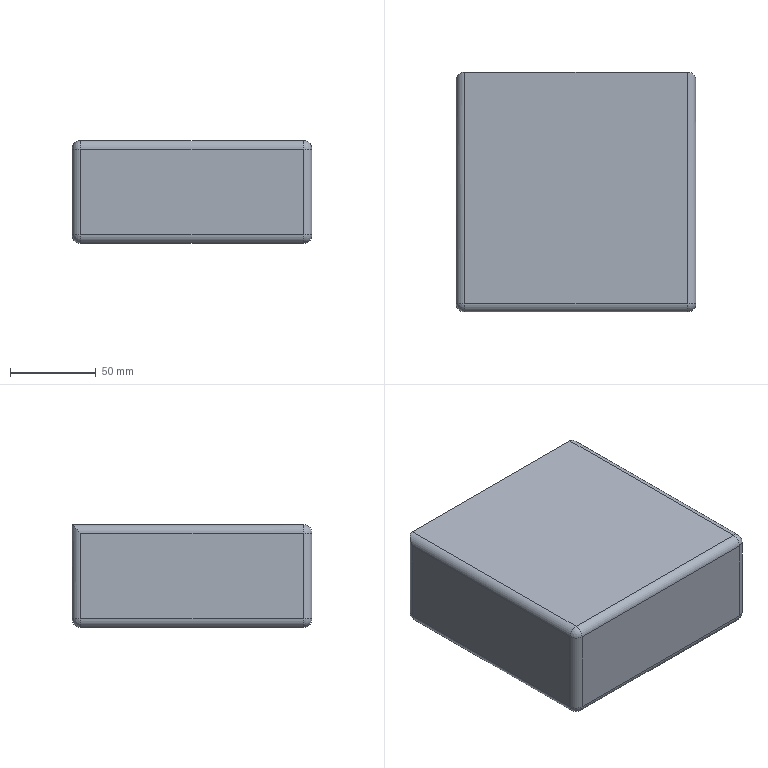Component | SolidWorks | ConnectingBlock-1 | 1 solid | 26 faces | box 140 x 140 x 60 mm | volume 1078498 mm3 | cylinder 13 | plane 7 | sphere 6 | commonest cylinder face diameters 10 x11 60 x2
build123d program:
from build123d import *

# Parameters (mm, degrees)
SKETCH1_W                 = 140
SKETCH1_H                 = 140
BOSS_EXTRUDE1_DEPTH       = 60
FILLET1_R                 = 5
SKETCH2_R                 = 30
REPAIR_RODENDSOCKET_DEPTH = 16.832


with BuildPart() as part:
    # Sketch1 → Boss-Extrude1 (new body)
    with BuildSketch(Plane(origin=(0, 0, -32.222), x_dir=(-1, 0, 0), z_dir=(0, 0, -1))):
        Rectangle(SKETCH1_W, SKETCH1_H)
    extrude(amount=-BOSS_EXTRUDE1_DEPTH)

    # Fillet1
    fillet1_edges = [part.edges().sort_by_distance(p)[0] for p in [
        (0, -70, 27.778),
        (-70, 0, 27.778),
        (0, -70, -32.222),
        (70, 0, -32.222),
        (0, 70, -32.222),
        (-70, 0, -32.222),
        (-70, -70, -2.222),
        (70, -70, -2.222),
        (70, 70, -2.222),
        (-70, 70, -2.222),
        (0, 70, 27.778),
    ]]
    fillet(fillet1_edges, radius=FILLET1_R)

    # Sketch2 → Repair_RodEndSocket (cut, symmetric)
    with BuildSketch(Plane.XY.offset(-16.832)):
        with Locations((0, 0)):
            Circle(SKETCH2_R)
    extrude(amount=REPAIR_RODENDSOCKET_DEPTH, both=True, mode=Mode.SUBTRACT)


solid = part.part

# Placed as in the assembly
solid = solid.moved(Location((-505.158, 870.769, 981.663), (0, 0, 90)))
STEP:
#1=CARTESIAN_POINT('',(-19.888,35.463,37.38));
#2=VERTEX_POINT('',#1);
#3=CARTESIAN_POINT('',(-19.888,33.101,37.38));
#4=VERTEX_POINT('',#3);
#5=CARTESIAN_POINT('',(-19.888,34.282,37.38));
#6=DIRECTION('',(0.,0.,-1.));
#7=DIRECTION('',(0.,-1.,0.));
#8=AXIS2_PLACEMENT_3D('',#5,#6,#7);
#9=CIRCLE('',#8,1.181);
#10=EDGE_CURVE('',#2,#4,#9,.T.);
#11=ORIENTED_EDGE('',*,*,#10,.T.);
#12=CARTESIAN_POINT('',(-19.888,33.101,38.648));
#13=VERTEX_POINT('',#12);
#14=CARTESIAN_POINT('',(-19.888,33.101,37.323));
#15=DIRECTION('',(0.,0.,1.));
#16=VECTOR('',#15,39.37);
#17=LINE('',#14,#16);
#18=EDGE_CURVE('',#4,#13,#17,.T.);
#19=ORIENTED_EDGE('',*,*,#18,.T.);
#20=CARTESIAN_POINT('',(-19.888,35.463,38.648));
#21=VERTEX_POINT('',#20);
#22=CARTESIAN_POINT('',(-19.888,34.282,38.648));
#23=DIRECTION('',(0.,0.,1.));
#24=DIRECTION('',(0.,1.,0.));
#25=AXIS2_PLACEMENT_3D('',#22,#23,#24);
#26=CIRCLE('',#25,1.181);
#27=EDGE_CURVE('',#13,#21,#26,.T.);
#28=ORIENTED_EDGE('',*,*,#27,.T.);
#29=CARTESIAN_POINT('',(-19.888,35.463,37.323));
#30=DIRECTION('',(0.,0.,1.));
#31=VECTOR('',#30,39.37);
#32=LINE('',#29,#31);
#33=EDGE_CURVE('',#2,#21,#32,.T.);
#34=ORIENTED_EDGE('',*,*,#33,.F.);
#35=EDGE_LOOP('',(#11,#19,#28,#34));
#36=FACE_OUTER_BOUND('',#35,.T.);
#37=CARTESIAN_POINT('',(-19.888,34.282,37.323));
#38=DIRECTION('',(0.,0.,1.));
#39=DIRECTION('',(0.,1.,0.));
#40=AXIS2_PLACEMENT_3D('',#37,#38,#39);
#41=CYLINDRICAL_SURFACE('',#40,1.181);
#42=ADVANCED_FACE('',(#36),#41,.F.);
#43=CARTESIAN_POINT('',(-22.447,31.526,37.576));
#44=VERTEX_POINT('',#43);
#45=CARTESIAN_POINT('',(-17.329,31.526,37.576));
#46=VERTEX_POINT('',#45);
#47=CARTESIAN_POINT('',(-17.132,31.526,37.576));
#48=DIRECTION('',(1.,0.,0.));
#49=VECTOR('',#48,39.37);
#50=LINE('',#47,#49);
#51=EDGE_CURVE('',#44,#46,#50,.T.);
#52=ORIENTED_EDGE('',*,*,#51,.T.);
#53=CARTESIAN_POINT('',(-17.329,31.526,39.545));
#54=VERTEX_POINT('',#53);
#55=CARTESIAN_POINT('',(-17.329,31.526,39.742));
#56=DIRECTION('',(0.,0.,1.));
#57=VECTOR('',#56,39.37);
#58=LINE('',#55,#57);
#59=EDGE_CURVE('',#46,#54,#58,.T.);
#60=ORIENTED_EDGE('',*,*,#59,.T.);
#61=CARTESIAN_POINT('',(-22.447,31.526,39.545));
#62=VERTEX_POINT('',#61);
#63=CARTESIAN_POINT('',(-22.644,31.526,39.545));
#64=DIRECTION('',(-1.,0.,0.));
#65=VECTOR('',#64,39.37);
#66=LINE('',#63,#65);
#67=EDGE_CURVE('',#54,#62,#66,.T.);
#68=ORIENTED_EDGE('',*,*,#67,.T.);
#69=CARTESIAN_POINT('',(-22.447,31.526,39.742));
#70=DIRECTION('',(0.,0.,-1.));
#71=VECTOR('',#70,39.37);
#72=LINE('',#69,#71);
#73=EDGE_CURVE('',#62,#44,#72,.T.);
#74=ORIENTED_EDGE('',*,*,#73,.T.);
#75=EDGE_LOOP('',(#52,#60,#68,#74));
#76=FACE_OUTER_BOUND('',#75,.T.);
#77=CARTESIAN_POINT('',(-17.132,31.526,39.742));
#78=DIRECTION('',(0.,-1.,0.));
#79=DIRECTION('',(0.,0.,1.));
#80=AXIS2_PLACEMENT_3D('',#77,#78,#79);
#81=PLANE('',#80);
#82=ADVANCED_FACE('',(#76),#81,.T.);
#83=CARTESIAN_POINT('',(-17.132,36.841,37.576));
#84=VERTEX_POINT('',#83);
#85=CARTESIAN_POINT('',(-17.132,36.841,39.545));
#86=VERTEX_POINT('',#85);
#87=CARTESIAN_POINT('',(-17.132,36.841,39.742));
#88=DIRECTION('',(0.,0.,1.));
#89=VECTOR('',#88,39.37);
#90=LINE('',#87,#89);
#91=EDGE_CURVE('',#84,#86,#90,.T.);
#92=ORIENTED_EDGE('',*,*,#91,.T.);
#93=CARTESIAN_POINT('',(-17.132,31.723,39.545));
#94=VERTEX_POINT('',#93);
#95=CARTESIAN_POINT('',(-17.132,31.526,39.545));
#96=DIRECTION('',(0.,-1.,0.));
#97=VECTOR('',#96,39.37);
#98=LINE('',#95,#97);
#99=EDGE_CURVE('',#86,#94,#98,.T.);
#100=ORIENTED_EDGE('',*,*,#99,.T.);
#101=CARTESIAN_POINT('',(-17.132,31.723,37.576));
#102=VERTEX_POINT('',#101);
#103=CARTESIAN_POINT('',(-17.132,31.723,39.742));
#104=DIRECTION('',(0.,0.,-1.));
#105=VECTOR('',#104,39.37);
#106=LINE('',#103,#105);
#107=EDGE_CURVE('',#94,#102,#106,.T.);
#108=ORIENTED_EDGE('',*,*,#107,.T.);
#109=CARTESIAN_POINT('',(-17.132,37.038,37.576));
#110=DIRECTION('',(0.,1.,0.));
#111=VECTOR('',#110,39.37);
#112=LINE('',#109,#111);
#113=EDGE_CURVE('',#102,#84,#112,.T.);
#114=ORIENTED_EDGE('',*,*,#113,.T.);
#115=EDGE_LOOP('',(#92,#100,#108,#114));
#116=FACE_OUTER_BOUND('',#115,.T.);
#117=CARTESIAN_POINT('',(-17.132,37.038,39.742));
#118=DIRECTION('',(1.,0.,0.));
#119=DIRECTION('',(0.,0.,-1.));
#120=AXIS2_PLACEMENT_3D('',#117,#118,#119);
#121=PLANE('',#120);
#122=ADVANCED_FACE('',(#116),#121,.T.);
#123=CARTESIAN_POINT('',(-22.447,37.038,39.742));
#124=VERTEX_POINT('',#123);
#125=CARTESIAN_POINT('',(-17.329,37.038,39.742));
#126=VERTEX_POINT('',#125);
#127=CARTESIAN_POINT('',(-22.644,37.038,39.742));
#128=DIRECTION('',(1.,0.,0.));
#129=VECTOR('',#128,39.37);
#130=LINE('',#127,#129);
#131=EDGE_CURVE('',#124,#126,#130,.T.);
#132=ORIENTED_EDGE('',*,*,#131,.T.);
#133=CARTESIAN_POINT('',(-17.329,37.038,37.576));
#134=VERTEX_POINT('',#133);
#135=CARTESIAN_POINT('',(-17.329,37.038,39.742));
#136=DIRECTION('',(0.,0.,-1.));
#137=VECTOR('',#136,39.37);
#138=LINE('',#135,#137);
#139=EDGE_CURVE('',#126,#134,#138,.T.);
#140=ORIENTED_EDGE('',*,*,#139,.T.);
#141=CARTESIAN_POINT('',(-22.447,37.038,37.576));
#142=VERTEX_POINT('',#141);
#143=CARTESIAN_POINT('',(-22.644,37.038,37.576));
#144=DIRECTION('',(-1.,0.,0.));
#145=VECTOR('',#144,39.37);
#146=LINE('',#143,#145);
#147=EDGE_CURVE('',#134,#142,#146,.T.);
#148=ORIENTED_EDGE('',*,*,#147,.T.);
#149=CARTESIAN_POINT('',(-22.447,37.038,39.742));
#150=DIRECTION('',(0.,0.,1.));
#151=VECTOR('',#150,39.37);
#152=LINE('',#149,#151);
#153=EDGE_CURVE('',#142,#124,#152,.T.);
#154=ORIENTED_EDGE('',*,*,#153,.T.);
#155=EDGE_LOOP('',(#132,#140,#148,#154));
#156=FACE_OUTER_BOUND('',#155,.T.);
#157=CARTESIAN_POINT('',(-22.644,37.038,39.742));
#158=DIRECTION('',(0.,1.,0.));
#159=DIRECTION('',(0.,0.,-1.));
#160=AXIS2_PLACEMENT_3D('',#157,#158,#159);
#161=PLANE('',#160);
#162=ADVANCED_FACE('',(#156),#161,.T.);
#163=CARTESIAN_POINT('',(-22.644,36.841,37.576));
#164=VERTEX_POINT('',#163);
#165=CARTESIAN_POINT('',(-22.644,31.723,37.576));
#166=VERTEX_POINT('',#165);
#167=CARTESIAN_POINT('',(-22.644,31.526,37.576));
#168=DIRECTION('',(0.,-1.,0.));
#169=VECTOR('',#168,39.37);
#170=LINE('',#167,#169);
#171=EDGE_CURVE('',#164,#166,#170,.T.);
#172=ORIENTED_EDGE('',*,*,#171,.T.);
#173=CARTESIAN_POINT('',(-22.644,31.723,39.545));
#174=VERTEX_POINT('',#173);
#175=CARTESIAN_POINT('',(-22.644,31.723,39.742));
#176=DIRECTION('',(0.,0.,1.));
#177=VECTOR('',#176,39.37);
#178=LINE('',#175,#177);
#179=EDGE_CURVE('',#166,#174,#178,.T.);
#180=ORIENTED_EDGE('',*,*,#179,.T.);
#181=CARTESIAN_POINT('',(-22.644,36.841,39.545));
#182=VERTEX_POINT('',#181);
#183=CARTESIAN_POINT('',(-22.644,37.038,39.545));
#184=DIRECTION('',(0.,1.,0.));
#185=VECTOR('',#184,39.37);
#186=LINE('',#183,#185);
#187=EDGE_CURVE('',#174,#182,#186,.T.);
#188=ORIENTED_EDGE('',*,*,#187,.T.);
#189=CARTESIAN_POINT('',(-22.644,36.841,39.742));
#190=DIRECTION('',(0.,0.,-1.));
#191=VECTOR('',#190,39.37);
#192=LINE('',#189,#191);
#193=EDGE_CURVE('',#182,#164,#192,.T.);
#194=ORIENTED_EDGE('',*,*,#193,.T.);
#195=EDGE_LOOP('',(#172,#180,#188,#194));
#196=FACE_OUTER_BOUND('',#195,.T.);
#197=CARTESIAN_POINT('',(-22.644,31.526,39.742));
#198=DIRECTION('',(-1.,0.,0.));
#199=DIRECTION('',(0.,0.,1.));
#200=AXIS2_PLACEMENT_3D('',#197,#198,#199);
#201=PLANE('',#200);
#202=ADVANCED_FACE('',(#196),#201,.T.);
#203=CARTESIAN_POINT('',(-22.447,31.723,39.742));
#204=VERTEX_POINT('',#203);
#205=CARTESIAN_POINT('',(-17.329,31.723,39.742));
#206=VERTEX_POINT('',#205);
#207=CARTESIAN_POINT('',(-17.132,31.723,39.742));
#208=DIRECTION('',(1.,0.,0.));
#209=VECTOR('',#208,39.37);
#210=LINE('',#207,#209);
#211=EDGE_CURVE('',#204,#206,#210,.T.);
#212=ORIENTED_EDGE('',*,*,#211,.T.);
#213=CARTESIAN_POINT('',(-17.329,37.038,39.742));
#214=DIRECTION('',(0.,1.,0.));
#215=VECTOR('',#214,39.37);
#216=LINE('',#213,#215);
#217=EDGE_CURVE('',#206,#126,#216,.T.);
#218=ORIENTED_EDGE('',*,*,#217,.T.);
#219=ORIENTED_EDGE('',*,*,#131,.F.);
#220=CARTESIAN_POINT('',(-22.447,31.526,39.742));
#221=DIRECTION('',(0.,-1.,0.));
#222=VECTOR('',#221,39.37);
#223=LINE('',#220,#222);
#224=EDGE_CURVE('',#124,#204,#223,.T.);
#225=ORIENTED_EDGE('',*,*,#224,.T.);
#226=EDGE_LOOP('',(#212,#218,#219,#225));
#227=FACE_OUTER_BOUND('',#226,.T.);
#228=CARTESIAN_POINT('',(-19.888,34.282,39.742));
#229=DIRECTION('',(0.,0.,-1.));
#230=DIRECTION('',(0.,-1.,0.));
#231=AXIS2_PLACEMENT_3D('',#228,#229,#230);
#232=PLANE('',#231);
#233=ADVANCED_FACE('',(#227),#232,.F.);
#234=ORIENTED_EDGE('',*,*,#10,.F.);
#235=CARTESIAN_POINT('',(-19.888,34.282,37.38));
#236=DIRECTION('',(0.,0.,-1.));
#237=DIRECTION('',(0.,-1.,0.));
#238=AXIS2_PLACEMENT_3D('',#235,#236,#237);
#239=CIRCLE('',#238,1.181);
#240=EDGE_CURVE('',#4,#2,#239,.T.);
#241=ORIENTED_EDGE('',*,*,#240,.F.);
#242=EDGE_LOOP('',(#234,#241));
#243=FACE_BOUND('',#242,.T.);
#244=CARTESIAN_POINT('',(-22.447,36.841,37.38));
#245=VERTEX_POINT('',#244);
#246=CARTESIAN_POINT('',(-17.329,36.841,37.38));
#247=VERTEX_POINT('',#246);
#248=CARTESIAN_POINT('',(-19.888,36.841,37.38));
#249=DIRECTION('',(1.,0.,0.));
#250=VECTOR('',#249,39.37);
#251=LINE('',#248,#250);
#252=EDGE_CURVE('',#245,#247,#251,.T.);
#253=ORIENTED_EDGE('',*,*,#252,.T.);
#254=CARTESIAN_POINT('',(-17.329,31.723,37.38));
#255=VERTEX_POINT('',#254);
#256=CARTESIAN_POINT('',(-17.329,34.282,37.38));
#257=DIRECTION('',(0.,-1.,0.));
#258=VECTOR('',#257,39.37);
#259=LINE('',#256,#258);
#260=EDGE_CURVE('',#247,#255,#259,.T.);
#261=ORIENTED_EDGE('',*,*,#260,.T.);
#262=CARTESIAN_POINT('',(-22.447,31.723,37.38));
#263=VERTEX_POINT('',#262);
#264=CARTESIAN_POINT('',(-19.888,31.723,37.38));
#265=DIRECTION('',(-1.,0.,0.));
#266=VECTOR('',#265,39.37);
#267=LINE('',#264,#266);
#268=EDGE_CURVE('',#255,#263,#267,.T.);
#269=ORIENTED_EDGE('',*,*,#268,.T.);
#270=CARTESIAN_POINT('',(-22.447,34.282,37.38));
#271=DIRECTION('',(0.,1.,0.));
#272=VECTOR('',#271,39.37);
#273=LINE('',#270,#272);
#274=EDGE_CURVE('',#263,#245,#273,.T.);
#275=ORIENTED_EDGE('',*,*,#274,.T.);
#276=EDGE_LOOP('',(#253,#261,#269,#275));
#277=FACE_OUTER_BOUND('',#276,.T.);
#278=CARTESIAN_POINT('',(-19.888,34.282,37.38));
#279=DIRECTION('',(0.,0.,-1.));
#280=DIRECTION('',(0.,-1.,0.));
#281=AXIS2_PLACEMENT_3D('',#278,#279,#280);
#282=PLANE('',#281);
#283=ADVANCED_FACE('',(#243,#277),#282,.T.);
#284=CARTESIAN_POINT('',(-22.447,31.723,37.576));
#285=DIRECTION('',(0.,-1.,0.));
#286=DIRECTION('',(0.,0.,1.));
#287=AXIS2_PLACEMENT_3D('',#284,#285,#286);
#288=CIRCLE('',#287,0.1969);
#289=EDGE_CURVE('',#166,#263,#288,.T.);
#290=ORIENTED_EDGE('',*,*,#289,.F.);
#291=ORIENTED_EDGE('',*,*,#171,.F.);
#292=CARTESIAN_POINT('',(-22.447,36.841,37.576));
#293=DIRECTION('',(0.,1.,0.));
#294=DIRECTION('',(0.,0.,-1.));
#295=AXIS2_PLACEMENT_3D('',#292,#293,#294);
#296=CIRCLE('',#295,0.1969);
#297=EDGE_CURVE('',#245,#164,#296,.T.);
#298=ORIENTED_EDGE('',*,*,#297,.F.);
#299=ORIENTED_EDGE('',*,*,#274,.F.);
#300=EDGE_LOOP('',(#290,#291,#298,#299));
#301=FACE_OUTER_BOUND('',#300,.T.);
#302=CARTESIAN_POINT('',(-22.447,34.282,37.576));
#303=DIRECTION('',(0.,1.,0.));
#304=DIRECTION('',(0.,0.,-1.));
#305=AXIS2_PLACEMENT_3D('',#302,#303,#304);
#306=CYLINDRICAL_SURFACE('',#305,0.1969);
#307=ADVANCED_FACE('',(#301),#306,.T.);
#308=CARTESIAN_POINT('',(-22.447,31.723,37.576));
#309=DIRECTION('',(0.,0.,1.));
#310=DIRECTION('',(0.,-1.,0.));
#311=AXIS2_PLACEMENT_3D('',#308,#309,#310);
#312=CIRCLE('',#311,0.1969);
#313=EDGE_CURVE('',#166,#44,#312,.T.);
#314=ORIENTED_EDGE('',*,*,#313,.F.);
#315=ORIENTED_EDGE('',*,*,#289,.T.);
#316=CARTESIAN_POINT('',(-22.447,31.723,37.576));
#317=DIRECTION('',(1.,0.,0.));
#318=DIRECTION('',(0.,0.,1.));
#319=AXIS2_PLACEMENT_3D('',#316,#317,#318);
#320=CIRCLE('',#319,0.1969);
#321=EDGE_CURVE('',#44,#263,#320,.T.);
#322=ORIENTED_EDGE('',*,*,#321,.F.);
#323=EDGE_LOOP('',(#314,#315,#322));
#324=FACE_OUTER_BOUND('',#323,.T.);
#325=CARTESIAN_POINT('',(-22.447,31.723,37.576));
#326=DIRECTION('',(-1.,0.,0.));
#327=DIRECTION('',(0.,1.,0.));
#328=AXIS2_PLACEMENT_3D('',#325,#326,#327);
#329=SPHERICAL_SURFACE('',#328,0.1969);
#330=ADVANCED_FACE('',(#324),#329,.T.);
#331=CARTESIAN_POINT('',(-22.447,36.841,37.576));
#332=DIRECTION('',(0.,0.,-1.));
#333=DIRECTION('',(0.,-1.,0.));
#334=AXIS2_PLACEMENT_3D('',#331,#332,#333);
#335=CIRCLE('',#334,0.1969);
#336=EDGE_CURVE('',#164,#142,#335,.T.);
#337=ORIENTED_EDGE('',*,*,#336,.F.);
#338=ORIENTED_EDGE('',*,*,#193,.F.);
#339=CARTESIAN_POINT('',(-22.447,37.038,39.742));
#340=CARTESIAN_POINT('',(-22.562,37.038,39.742));
#341=CARTESIAN_POINT('',(-22.644,36.957,39.66));
#342=CARTESIAN_POINT('',(-22.644,36.841,39.545));
#343=(BOUNDED_CURVE()B_SPLINE_CURVE(3,(#339,#340,#341,#342),.UNSPECIFIED.,.F.,.F.)B_SPLINE_CURVE_WITH_KNOTS((4,4),(3.142,4.712),.UNSPECIFIED.)CURVE()GEOMETRIC_REPRESENTATION_ITEM()RATIONAL_B_SPLINE_CURVE((1.,0.8047,0.8047,1.))REPRESENTATION_ITEM(''));
#344=EDGE_CURVE('',#124,#182,#343,.T.);
#345=ORIENTED_EDGE('',*,*,#344,.F.);
#346=ORIENTED_EDGE('',*,*,#153,.F.);
#347=EDGE_LOOP('',(#337,#338,#345,#346));
#348=FACE_OUTER_BOUND('',#347,.T.);
#349=CARTESIAN_POINT('',(-22.447,36.841,39.742));
#350=DIRECTION('',(0.,0.,-1.));
#351=DIRECTION('',(0.,-1.,0.));
#352=AXIS2_PLACEMENT_3D('',#349,#350,#351);
#353=CYLINDRICAL_SURFACE('',#352,0.1969);
#354=ADVANCED_FACE('',(#348),#353,.T.);
#355=ORIENTED_EDGE('',*,*,#297,.T.);
#356=ORIENTED_EDGE('',*,*,#336,.T.);
#357=CARTESIAN_POINT('',(-22.447,36.841,37.576));
#358=DIRECTION('',(1.,0.,0.));
#359=DIRECTION('',(0.,0.,1.));
#360=AXIS2_PLACEMENT_3D('',#357,#358,#359);
#361=CIRCLE('',#360,0.1969);
#362=EDGE_CURVE('',#245,#142,#361,.T.);
#363=ORIENTED_EDGE('',*,*,#362,.F.);
#364=EDGE_LOOP('',(#355,#356,#363));
#365=FACE_OUTER_BOUND('',#364,.T.);
#366=CARTESIAN_POINT('',(-22.447,36.841,37.576));
#367=DIRECTION('',(-1.,0.,0.));
#368=DIRECTION('',(0.,1.,0.));
#369=AXIS2_PLACEMENT_3D('',#366,#367,#368);
#370=SPHERICAL_SURFACE('',#369,0.1969);
#371=ADVANCED_FACE('',(#365),#370,.T.);
#372=ORIENTED_EDGE('',*,*,#321,.T.);
#373=ORIENTED_EDGE('',*,*,#268,.F.);
#374=CARTESIAN_POINT('',(-17.329,31.723,37.576));
#375=DIRECTION('',(1.,0.,0.));
#376=DIRECTION('',(0.,0.,-1.));
#377=AXIS2_PLACEMENT_3D('',#374,#375,#376);
#378=CIRCLE('',#377,0.1969);
#379=EDGE_CURVE('',#46,#255,#378,.T.);
#380=ORIENTED_EDGE('',*,*,#379,.F.);
#381=ORIENTED_EDGE('',*,*,#51,.F.);
#382=EDGE_LOOP('',(#372,#373,#380,#381));
#383=FACE_OUTER_BOUND('',#382,.T.);
#384=CARTESIAN_POINT('',(-19.888,31.723,37.576));
#385=DIRECTION('',(-1.,0.,0.));
#386=DIRECTION('',(0.,0.,1.));
#387=AXIS2_PLACEMENT_3D('',#384,#385,#386);
#388=CYLINDRICAL_SURFACE('',#387,0.1969);
#389=ADVANCED_FACE('',(#383),#388,.T.);
#390=ORIENTED_EDGE('',*,*,#313,.T.);
#391=ORIENTED_EDGE('',*,*,#73,.F.);
#392=CARTESIAN_POINT('',(-22.447,31.723,39.545));
#393=DIRECTION('',(0.,0.,1.));
#394=DIRECTION('',(0.,1.,0.));
#395=AXIS2_PLACEMENT_3D('',#392,#393,#394);
#396=CIRCLE('',#395,0.1969);
#397=EDGE_CURVE('',#174,#62,#396,.T.);
#398=ORIENTED_EDGE('',*,*,#397,.F.);
#399=ORIENTED_EDGE('',*,*,#179,.F.);
#400=EDGE_LOOP('',(#390,#391,#398,#399));
#401=FACE_OUTER_BOUND('',#400,.T.);
#402=CARTESIAN_POINT('',(-22.447,31.723,39.742));
#403=DIRECTION('',(0.,0.,-1.));
#404=DIRECTION('',(0.,-1.,0.));
#405=AXIS2_PLACEMENT_3D('',#402,#403,#404);
#406=CYLINDRICAL_SURFACE('',#405,0.1969);
#407=ADVANCED_FACE('',(#401),#406,.T.);
#408=ORIENTED_EDGE('',*,*,#344,.T.);
#409=ORIENTED_EDGE('',*,*,#187,.F.);
#410=CARTESIAN_POINT('',(-22.447,31.723,39.545));
#411=DIRECTION('',(0.,-1.,0.));
#412=DIRECTION('',(0.,0.,1.));
#413=AXIS2_PLACEMENT_3D('',#410,#411,#412);
#414=CIRCLE('',#413,0.1969);
#415=EDGE_CURVE('',#204,#174,#414,.T.);
#416=ORIENTED_EDGE('',*,*,#415,.F.);
#417=ORIENTED_EDGE('',*,*,#224,.F.);
#418=EDGE_LOOP('',(#408,#409,#416,#417));
#419=FACE_OUTER_BOUND('',#418,.T.);
#420=CARTESIAN_POINT('',(-22.447,31.526,39.545));
#421=DIRECTION('',(0.,-1.,0.));
#422=DIRECTION('',(0.,0.,1.));
#423=AXIS2_PLACEMENT_3D('',#420,#421,#422);
#424=CYLINDRICAL_SURFACE('',#423,0.1969);
#425=ADVANCED_FACE('',(#419),#424,.T.);
#426=ORIENTED_EDGE('',*,*,#362,.T.);
#427=ORIENTED_EDGE('',*,*,#147,.F.);
#428=CARTESIAN_POINT('',(-17.329,36.841,37.576));
#429=DIRECTION('',(1.,0.,0.));
#430=DIRECTION('',(0.,0.,-1.));
#431=AXIS2_PLACEMENT_3D('',#428,#429,#430);
#432=CIRCLE('',#431,0.1969);
#433=EDGE_CURVE('',#247,#134,#432,.T.);
#434=ORIENTED_EDGE('',*,*,#433,.F.);
#435=ORIENTED_EDGE('',*,*,#252,.F.);
#436=EDGE_LOOP('',(#426,#427,#434,#435));
#437=FACE_OUTER_BOUND('',#436,.T.);
#438=CARTESIAN_POINT('',(-19.888,36.841,37.576));
#439=DIRECTION('',(1.,0.,0.));
#440=DIRECTION('',(0.,0.,-1.));
#441=AXIS2_PLACEMENT_3D('',#438,#439,#440);
#442=CYLINDRICAL_SURFACE('',#441,0.1969);
#443=ADVANCED_FACE('',(#437),#442,.T.);
#444=CARTESIAN_POINT('',(-17.329,31.723,37.576));
#445=DIRECTION('',(0.,-1.,0.));
#446=DIRECTION('',(0.,0.,1.));
#447=AXIS2_PLACEMENT_3D('',#444,#445,#446);
#448=CIRCLE('',#447,0.1969);
#449=EDGE_CURVE('',#255,#102,#448,.T.);
#450=ORIENTED_EDGE('',*,*,#449,.F.);
#451=ORIENTED_EDGE('',*,*,#260,.F.);
#452=CARTESIAN_POINT('',(-17.329,36.841,37.576));
#453=DIRECTION('',(0.,1.,0.));
#454=DIRECTION('',(0.,0.,-1.));
#455=AXIS2_PLACEMENT_3D('',#452,#453,#454);
#456=CIRCLE('',#455,0.1969);
#457=EDGE_CURVE('',#84,#247,#456,.T.);
#458=ORIENTED_EDGE('',*,*,#457,.F.);
#459=ORIENTED_EDGE('',*,*,#113,.F.);
#460=EDGE_LOOP('',(#450,#451,#458,#459));
#461=FACE_OUTER_BOUND('',#460,.T.);
#462=CARTESIAN_POINT('',(-17.329,34.282,37.576));
#463=DIRECTION('',(0.,-1.,0.));
#464=DIRECTION('',(0.,0.,1.));
#465=AXIS2_PLACEMENT_3D('',#462,#463,#464);
#466=CYLINDRICAL_SURFACE('',#465,0.1969);
#467=ADVANCED_FACE('',(#461),#466,.T.);
#468=ORIENTED_EDGE('',*,*,#379,.T.);
#469=ORIENTED_EDGE('',*,*,#449,.T.);
#470=CARTESIAN_POINT('',(-17.329,31.723,37.576));
#471=DIRECTION('',(0.,0.,1.));
#472=DIRECTION('',(0.,-1.,0.));
#473=AXIS2_PLACEMENT_3D('',#470,#471,#472);
#474=CIRCLE('',#473,0.1969);
#475=EDGE_CURVE('',#46,#102,#474,.T.);
#476=ORIENTED_EDGE('',*,*,#475,.F.);
#477=EDGE_LOOP('',(#468,#469,#476));
#478=FACE_OUTER_BOUND('',#477,.T.);
#479=CARTESIAN_POINT('',(-17.329,31.723,37.576));
#480=DIRECTION('',(-1.,0.,0.));
#481=DIRECTION('',(0.,1.,0.));
#482=AXIS2_PLACEMENT_3D('',#479,#480,#481);
#483=SPHERICAL_SURFACE('',#482,0.1969);
#484=ADVANCED_FACE('',(#478),#483,.T.);
#485=ORIENTED_EDGE('',*,*,#415,.T.);
#486=ORIENTED_EDGE('',*,*,#397,.T.);
#487=CARTESIAN_POINT('',(-22.447,31.723,39.545));
#488=DIRECTION('',(1.,0.,0.));
#489=DIRECTION('',(0.,0.,1.));
#490=AXIS2_PLACEMENT_3D('',#487,#488,#489);
#491=CIRCLE('',#490,0.1969);
#492=EDGE_CURVE('',#204,#62,#491,.T.);
#493=ORIENTED_EDGE('',*,*,#492,.F.);
#494=EDGE_LOOP('',(#485,#486,#493));
#495=FACE_OUTER_BOUND('',#494,.T.);
#496=CARTESIAN_POINT('',(-22.447,31.723,39.545));
#497=DIRECTION('',(-1.,0.,0.));
#498=DIRECTION('',(0.,1.,0.));
#499=AXIS2_PLACEMENT_3D('',#496,#497,#498);
#500=SPHERICAL_SURFACE('',#499,0.1969);
#501=ADVANCED_FACE('',(#495),#500,.T.);
#502=ORIENTED_EDGE('',*,*,#457,.T.);
#503=ORIENTED_EDGE('',*,*,#433,.T.);
#504=CARTESIAN_POINT('',(-17.329,36.841,37.576));
#505=DIRECTION('',(0.,0.,1.));
#506=DIRECTION('',(0.,-1.,0.));
#507=AXIS2_PLACEMENT_3D('',#504,#505,#506);
#508=CIRCLE('',#507,0.1969);
#509=EDGE_CURVE('',#84,#134,#508,.T.);
#510=ORIENTED_EDGE('',*,*,#509,.F.);
#511=EDGE_LOOP('',(#502,#503,#510));
#512=FACE_OUTER_BOUND('',#511,.T.);
#513=CARTESIAN_POINT('',(-17.329,36.841,37.576));
#514=DIRECTION('',(-1.,0.,0.));
#515=DIRECTION('',(0.,1.,0.));
#516=AXIS2_PLACEMENT_3D('',#513,#514,#515);
#517=SPHERICAL_SURFACE('',#516,0.1969);
#518=ADVANCED_FACE('',(#512),#517,.T.);
#519=ORIENTED_EDGE('',*,*,#475,.T.);
#520=ORIENTED_EDGE('',*,*,#107,.F.);
#521=CARTESIAN_POINT('',(-17.329,31.723,39.545));
#522=DIRECTION('',(0.,0.,1.));
#523=DIRECTION('',(0.,1.,0.));
#524=AXIS2_PLACEMENT_3D('',#521,#522,#523);
#525=CIRCLE('',#524,0.1969);
#526=EDGE_CURVE('',#54,#94,#525,.T.);
#527=ORIENTED_EDGE('',*,*,#526,.F.);
#528=ORIENTED_EDGE('',*,*,#59,.F.);
#529=EDGE_LOOP('',(#519,#520,#527,#528));
#530=FACE_OUTER_BOUND('',#529,.T.);
#531=CARTESIAN_POINT('',(-17.329,31.723,39.742));
#532=DIRECTION('',(0.,0.,-1.));
#533=DIRECTION('',(0.,-1.,0.));
#534=AXIS2_PLACEMENT_3D('',#531,#532,#533);
#535=CYLINDRICAL_SURFACE('',#534,0.1969);
#536=ADVANCED_FACE('',(#530),#535,.T.);
#537=ORIENTED_EDGE('',*,*,#492,.T.);
#538=ORIENTED_EDGE('',*,*,#67,.F.);
#539=CARTESIAN_POINT('',(-17.329,31.723,39.545));
#540=DIRECTION('',(1.,0.,0.));
#541=DIRECTION('',(0.,0.,-1.));
#542=AXIS2_PLACEMENT_3D('',#539,#540,#541);
#543=CIRCLE('',#542,0.1969);
#544=EDGE_CURVE('',#206,#54,#543,.T.);
#545=ORIENTED_EDGE('',*,*,#544,.F.);
#546=ORIENTED_EDGE('',*,*,#211,.F.);
#547=EDGE_LOOP('',(#537,#538,#545,#546));
#548=FACE_OUTER_BOUND('',#547,.T.);
#549=CARTESIAN_POINT('',(-17.132,31.723,39.545));
#550=DIRECTION('',(1.,0.,0.));
#551=DIRECTION('',(0.,0.,-1.));
#552=AXIS2_PLACEMENT_3D('',#549,#550,#551);
#553=CYLINDRICAL_SURFACE('',#552,0.1969);
#554=ADVANCED_FACE('',(#548),#553,.T.);
#555=ORIENTED_EDGE('',*,*,#509,.T.);
#556=ORIENTED_EDGE('',*,*,#139,.F.);
#557=CARTESIAN_POINT('',(-17.132,36.841,39.545));
#558=CARTESIAN_POINT('',(-17.132,36.957,39.66));
#559=CARTESIAN_POINT('',(-17.214,37.038,39.742));
#560=CARTESIAN_POINT('',(-17.329,37.038,39.742));
#561=(BOUNDED_CURVE()B_SPLINE_CURVE(3,(#557,#558,#559,#560),.UNSPECIFIED.,.F.,.F.)B_SPLINE_CURVE_WITH_KNOTS((4,4),(1.571,3.142),.UNSPECIFIED.)CURVE()GEOMETRIC_REPRESENTATION_ITEM()RATIONAL_B_SPLINE_CURVE((1.,0.8047,0.8047,1.))REPRESENTATION_ITEM(''));
#562=EDGE_CURVE('',#86,#126,#561,.T.);
#563=ORIENTED_EDGE('',*,*,#562,.F.);
#564=ORIENTED_EDGE('',*,*,#91,.F.);
#565=EDGE_LOOP('',(#555,#556,#563,#564));
#566=FACE_OUTER_BOUND('',#565,.T.);
#567=CARTESIAN_POINT('',(-17.329,36.841,39.742));
#568=DIRECTION('',(0.,0.,-1.));
#569=DIRECTION('',(0.,-1.,0.));
#570=AXIS2_PLACEMENT_3D('',#567,#568,#569);
#571=CYLINDRICAL_SURFACE('',#570,0.1969);
#572=ADVANCED_FACE('',(#566),#571,.T.);
#573=ORIENTED_EDGE('',*,*,#544,.T.);
#574=ORIENTED_EDGE('',*,*,#526,.T.);
#575=CARTESIAN_POINT('',(-17.329,31.723,39.545));
#576=DIRECTION('',(0.,1.,0.));
#577=DIRECTION('',(0.,0.,1.));
#578=AXIS2_PLACEMENT_3D('',#575,#576,#577);
#579=CIRCLE('',#578,0.1969);
#580=EDGE_CURVE('',#206,#94,#579,.T.);
#581=ORIENTED_EDGE('',*,*,#580,.F.);
#582=EDGE_LOOP('',(#573,#574,#581));
#583=FACE_OUTER_BOUND('',#582,.T.);
#584=CARTESIAN_POINT('',(-17.329,31.723,39.545));
#585=DIRECTION('',(-1.,0.,0.));
#586=DIRECTION('',(0.,1.,0.));
#587=AXIS2_PLACEMENT_3D('',#584,#585,#586);
#588=SPHERICAL_SURFACE('',#587,0.1969);
#589=ADVANCED_FACE('',(#583),#588,.T.);
#590=ORIENTED_EDGE('',*,*,#562,.T.);
#591=ORIENTED_EDGE('',*,*,#217,.F.);
#592=ORIENTED_EDGE('',*,*,#580,.T.);
#593=ORIENTED_EDGE('',*,*,#99,.F.);
#594=EDGE_LOOP('',(#590,#591,#592,#593));
#595=FACE_OUTER_BOUND('',#594,.T.);
#596=CARTESIAN_POINT('',(-17.329,37.038,39.545));
#597=DIRECTION('',(0.,1.,0.));
#598=DIRECTION('',(0.,0.,-1.));
#599=AXIS2_PLACEMENT_3D('',#596,#597,#598);
#600=CYLINDRICAL_SURFACE('',#599,0.1969);
#601=ADVANCED_FACE('',(#595),#600,.T.);
#602=ORIENTED_EDGE('',*,*,#18,.F.);
#603=ORIENTED_EDGE('',*,*,#240,.T.);
#604=ORIENTED_EDGE('',*,*,#33,.T.);
#605=CARTESIAN_POINT('',(-19.888,34.282,38.648));
#606=DIRECTION('',(0.,0.,1.));
#607=DIRECTION('',(0.,1.,0.));
#608=AXIS2_PLACEMENT_3D('',#605,#606,#607);
#609=CIRCLE('',#608,1.181);
#610=EDGE_CURVE('',#21,#13,#609,.T.);
#611=ORIENTED_EDGE('',*,*,#610,.T.);
#612=EDGE_LOOP('',(#602,#603,#604,#611));
#613=FACE_OUTER_BOUND('',#612,.T.);
#614=CARTESIAN_POINT('',(-19.888,34.282,37.323));
#615=DIRECTION('',(0.,0.,1.));
#616=DIRECTION('',(0.,1.,0.));
#617=AXIS2_PLACEMENT_3D('',#614,#615,#616);
#618=CYLINDRICAL_SURFACE('',#617,1.181);
#619=ADVANCED_FACE('',(#613),#618,.F.);
#620=ORIENTED_EDGE('',*,*,#610,.F.);
#621=ORIENTED_EDGE('',*,*,#27,.F.);
#622=EDGE_LOOP('',(#620,#621));
#623=FACE_OUTER_BOUND('',#622,.T.);
#624=CARTESIAN_POINT('',(-19.888,34.282,38.648));
#625=DIRECTION('',(0.,0.,1.));
#626=DIRECTION('',(0.,1.,0.));
#627=AXIS2_PLACEMENT_3D('',#624,#625,#626);
#628=PLANE('',#627);
#629=ADVANCED_FACE('',(#623),#628,.F.);
#630=CLOSED_SHELL('',(#42,#82,#122,#162,#202,#233,#283,#307,#330,#354,#371,#389,#407,#425,#443,#467,#484,#501,#518,#536,#554,#572,#589,#601,#619,#629));
#631=MANIFOLD_SOLID_BREP('',#630);
#632=CARTESIAN_POINT('',(0.,0.,0.));
#633=DIRECTION('',(0.,0.,1.));
#634=DIRECTION('',(1.,0.,0.));
#635=AXIS2_PLACEMENT_3D('',#632,#633,#634);
#636=(LENGTH_UNIT()NAMED_UNIT(*)SI_UNIT($,.METRE.));
#637=LENGTH_MEASURE_WITH_UNIT(LENGTH_MEASURE(0.0254),#636);
#638=DIMENSIONAL_EXPONENTS(1.,0.,0.,0.,0.,0.,0.);
#639=(CONVERSION_BASED_UNIT('',#637)LENGTH_UNIT()NAMED_UNIT(#638));
#640=UNCERTAINTY_MEASURE_WITH_UNIT(LENGTH_MEASURE(0.00001),#639,'','');
#641=(NAMED_UNIT(*)PLANE_ANGLE_UNIT()SI_UNIT($,.RADIAN.));
#642=(NAMED_UNIT(*)SI_UNIT($,.STERADIAN.)SOLID_ANGLE_UNIT());
#643=(GEOMETRIC_REPRESENTATION_CONTEXT(3)GLOBAL_UNCERTAINTY_ASSIGNED_CONTEXT((#640))GLOBAL_UNIT_ASSIGNED_CONTEXT((#639,#641,#642))REPRESENTATION_CONTEXT('',''));
#644=ADVANCED_BREP_SHAPE_REPRESENTATION('',(#631,#635),#643);
#645=COLOUR_RGB('',0.7922,0.8196,0.9333);
#646=FILL_AREA_STYLE_COLOUR('',#645);
#647=FILL_AREA_STYLE('',(#646));
#648=SURFACE_STYLE_FILL_AREA(#647);
#649=SURFACE_SIDE_STYLE('',(#648));
#650=SURFACE_STYLE_USAGE(.BOTH.,#649);
#651=PRESENTATION_STYLE_ASSIGNMENT((#650));
#652=STYLED_ITEM('',(#651),#631);
#653=PRESENTATION_LAYER_ASSIGNMENT('','',(#652));
#654=(LENGTH_UNIT()NAMED_UNIT(*)SI_UNIT($,.METRE.));
#655=LENGTH_MEASURE_WITH_UNIT(LENGTH_MEASURE(0.0254),#654);
#656=DIMENSIONAL_EXPONENTS(1.,0.,0.,0.,0.,0.,0.);
#657=(CONVERSION_BASED_UNIT('',#655)LENGTH_UNIT()NAMED_UNIT(#656));
#658=UNCERTAINTY_MEASURE_WITH_UNIT(LENGTH_MEASURE(0.00001),#657,'','');
#659=(NAMED_UNIT(*)PLANE_ANGLE_UNIT()SI_UNIT($,.RADIAN.));
#660=(NAMED_UNIT(*)SI_UNIT($,.STERADIAN.)SOLID_ANGLE_UNIT());
#661=(GEOMETRIC_REPRESENTATION_CONTEXT(3)GLOBAL_UNCERTAINTY_ASSIGNED_CONTEXT((#658))GLOBAL_UNIT_ASSIGNED_CONTEXT((#657,#659,#660))REPRESENTATION_CONTEXT('',''));
#662=MECHANICAL_DESIGN_GEOMETRIC_PRESENTATION_REPRESENTATION('',(#652),#661);